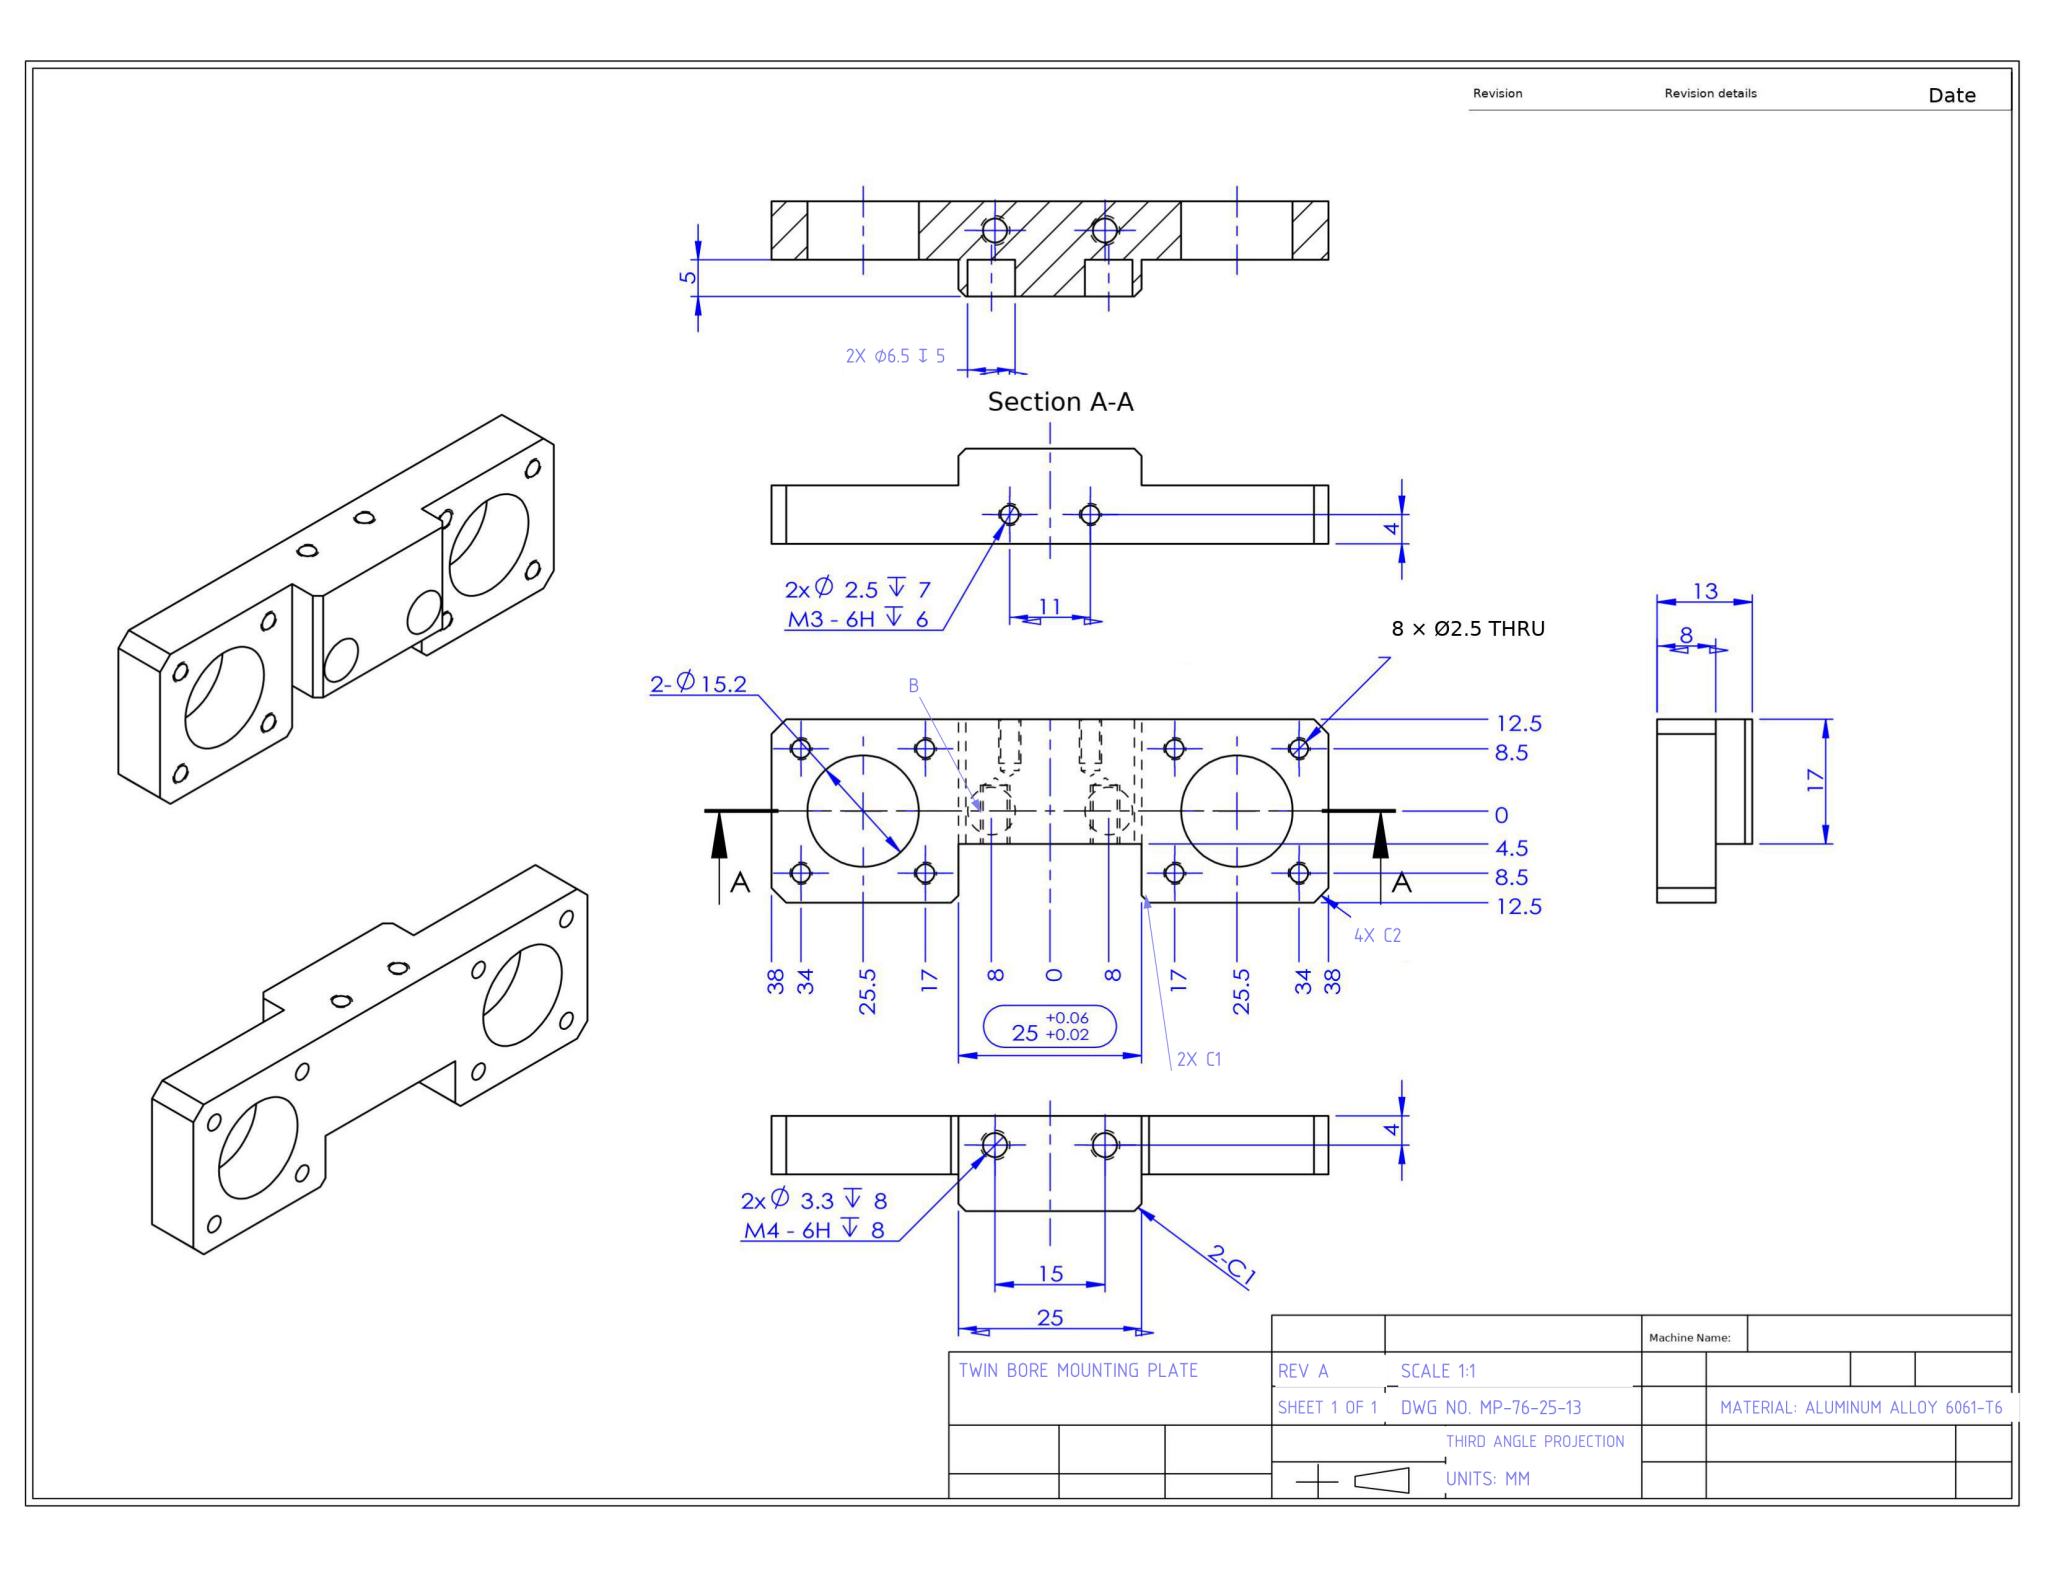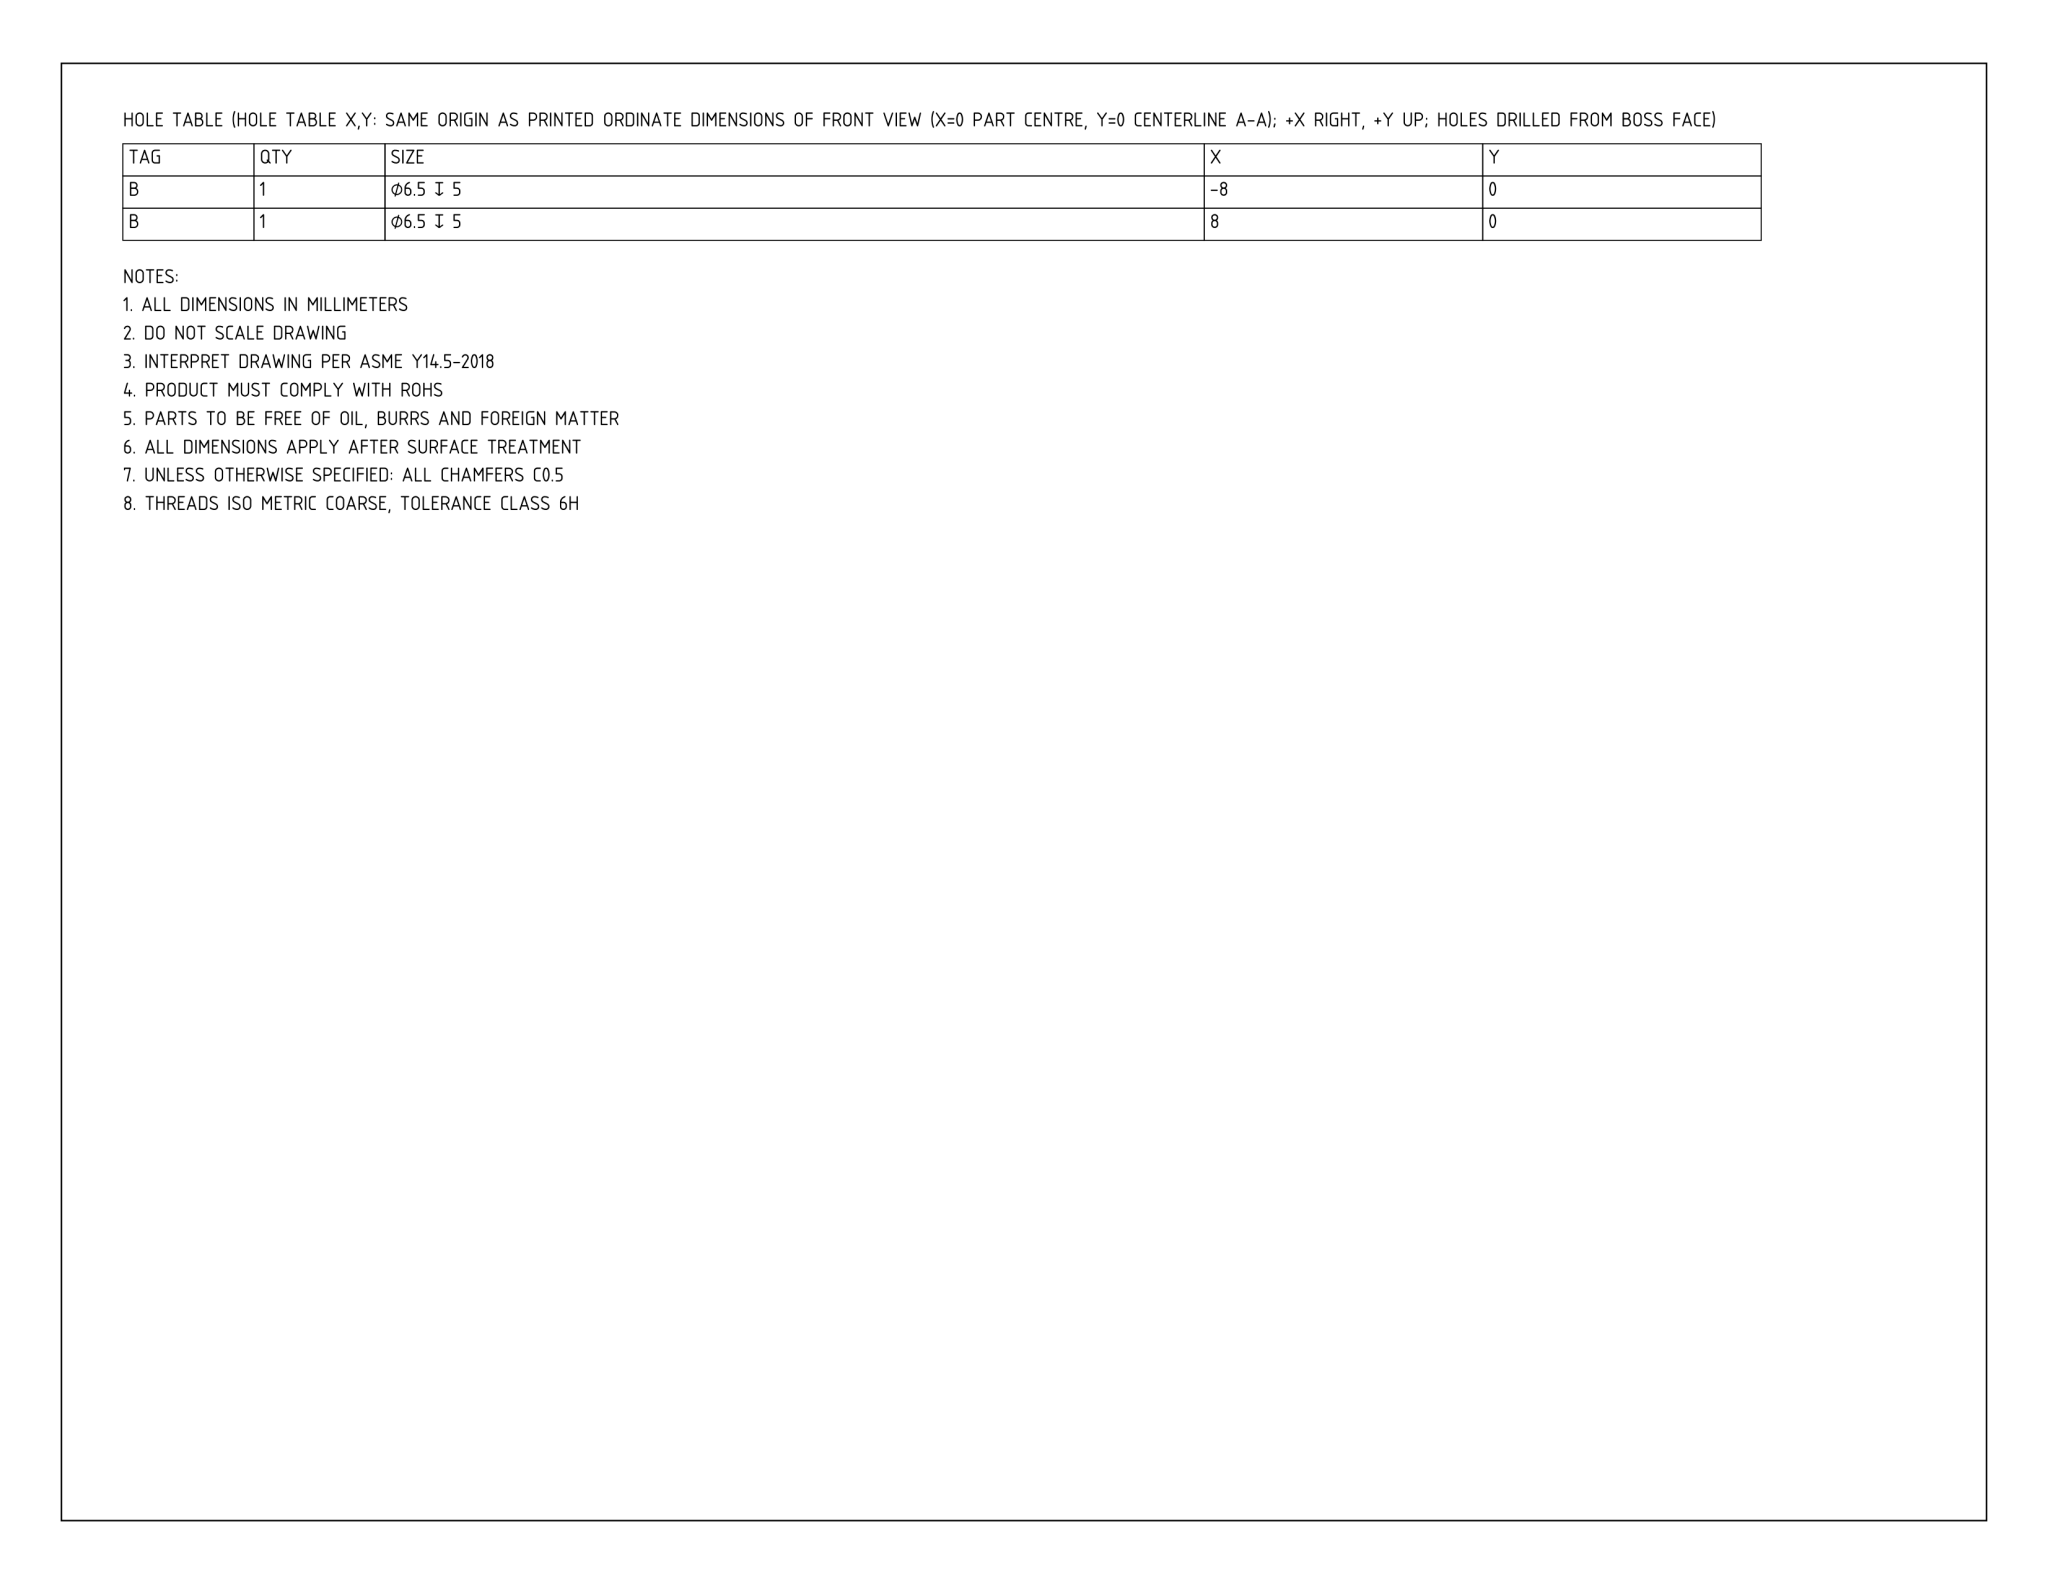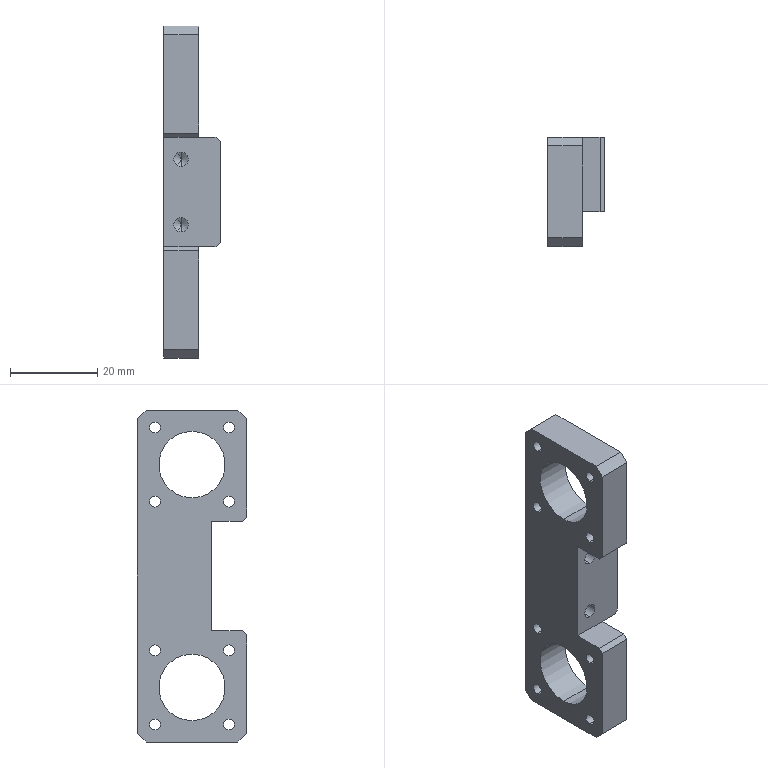Part | NX | mm | 1 solid | 64 faces | box 13 x 25 x 76 mm | volume 11873 mm3 | cylinder 32 | plane 24 | cone 8 | commonest cylinder face diameters 2.5 x20 6.5 x4 3.3 x4 15.2 x4